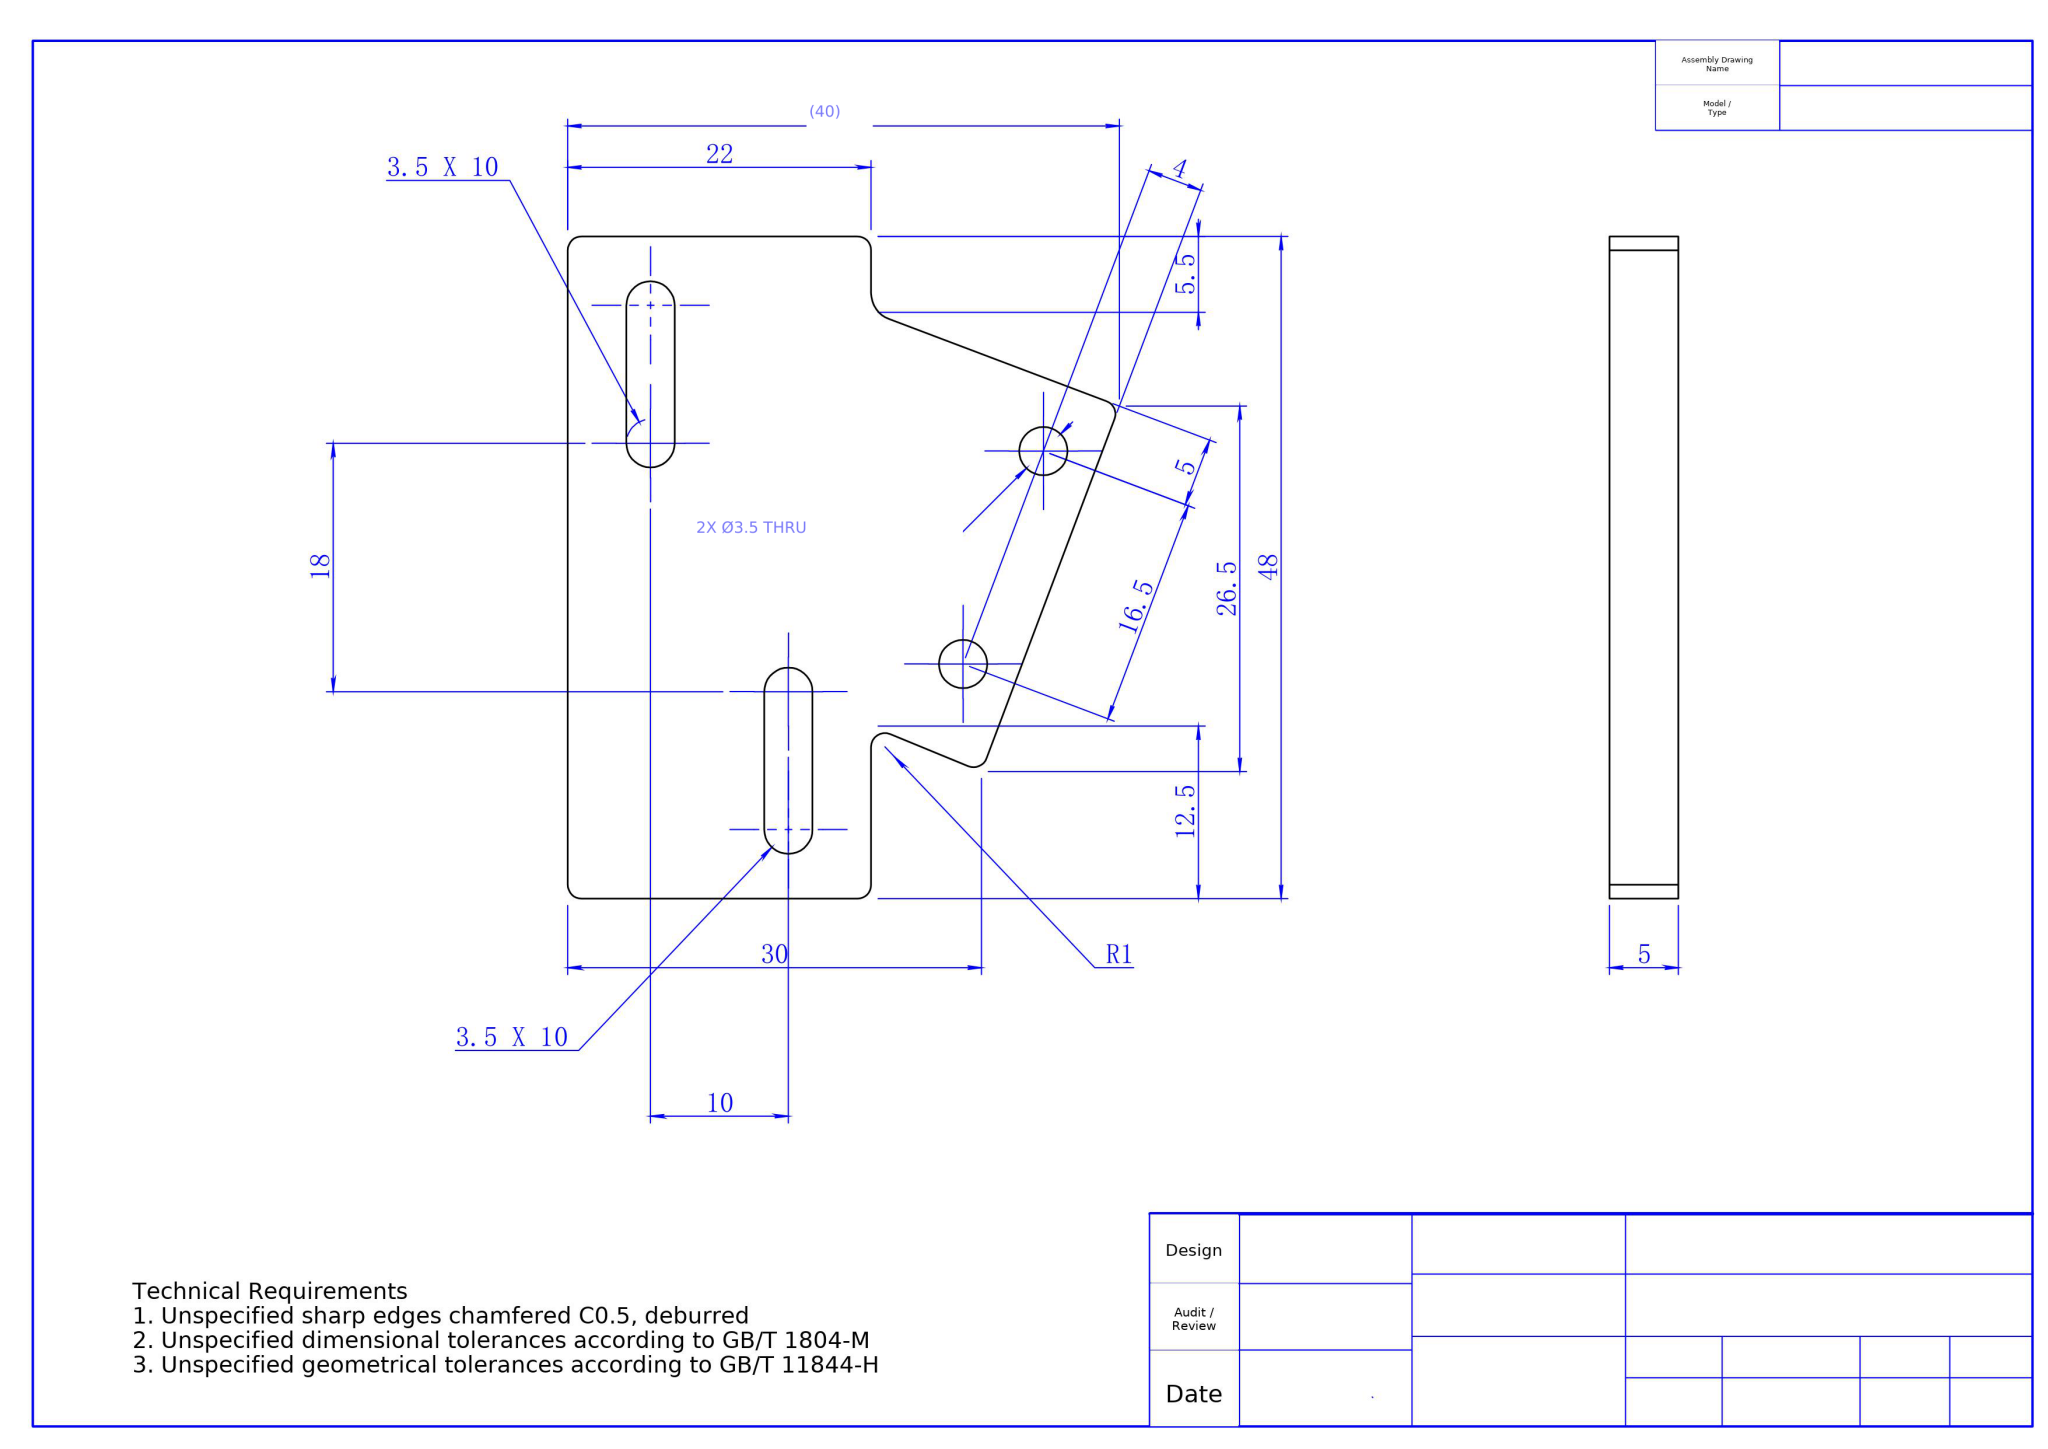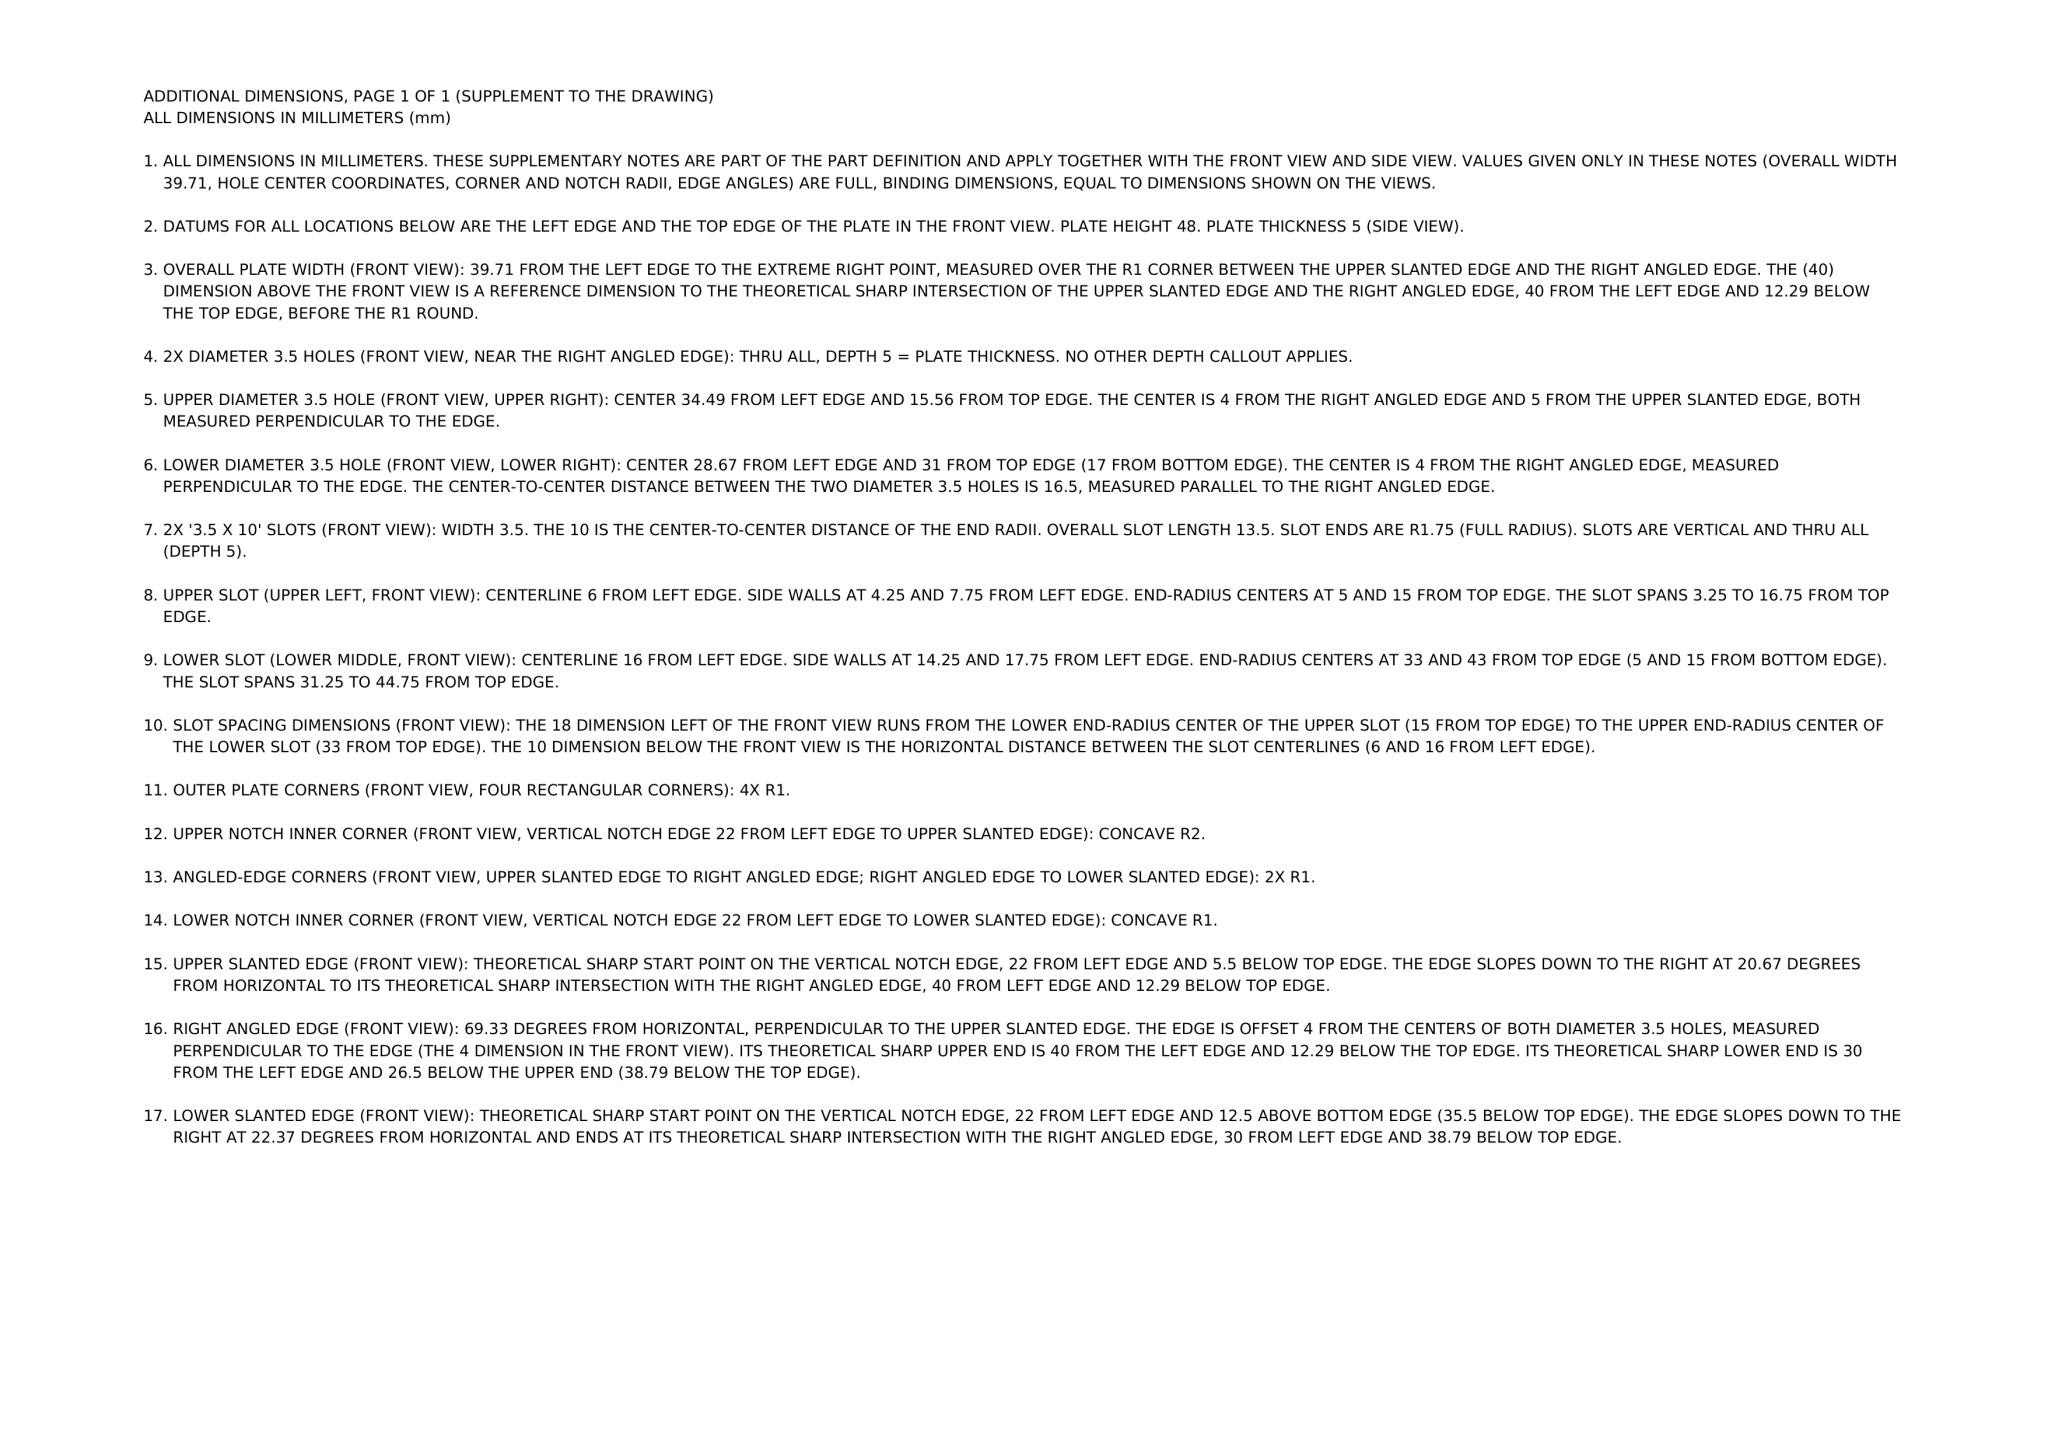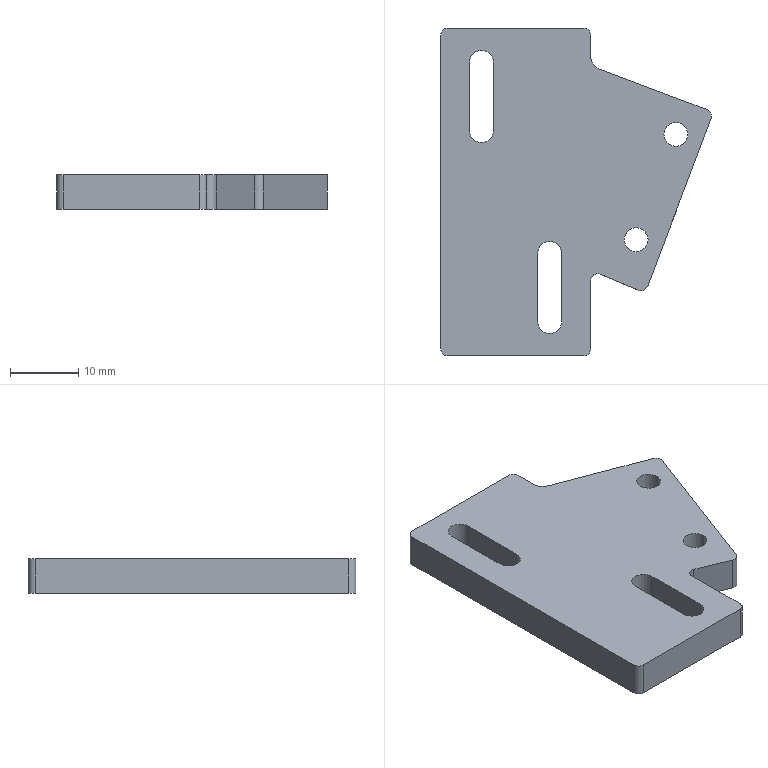Part | NX | mm | 1 solid | 31 faces | box 39.71 x 48 x 5 mm | volume 6698 mm3 | cylinder 17 | plane 14 | commonest cylinder face diameters 3.5 x8 2 x8 4 x1